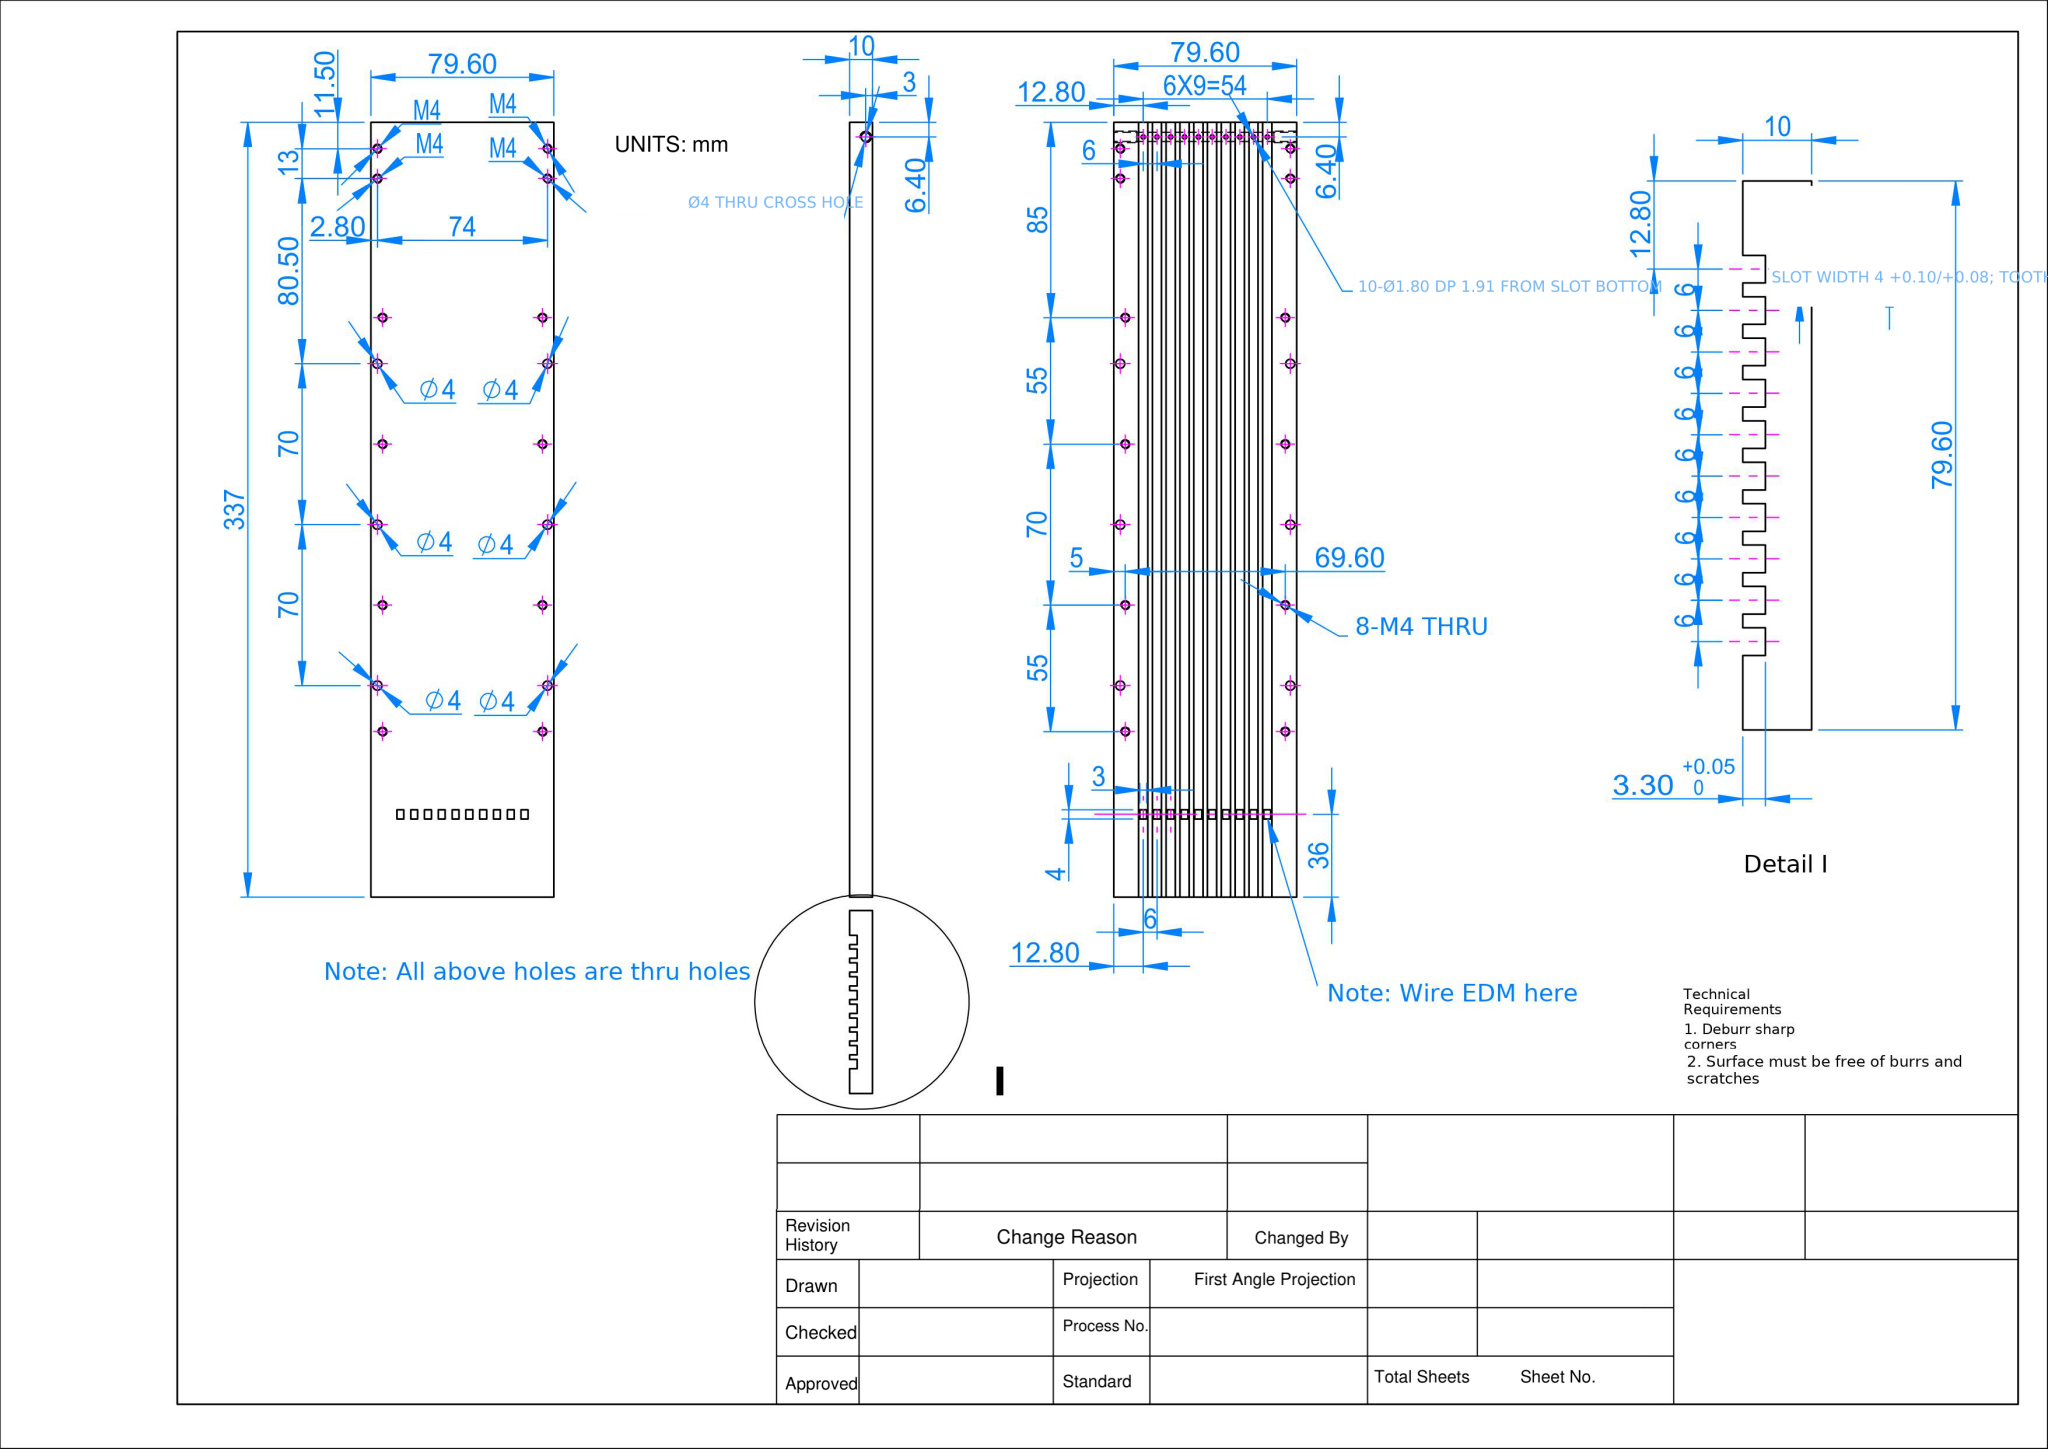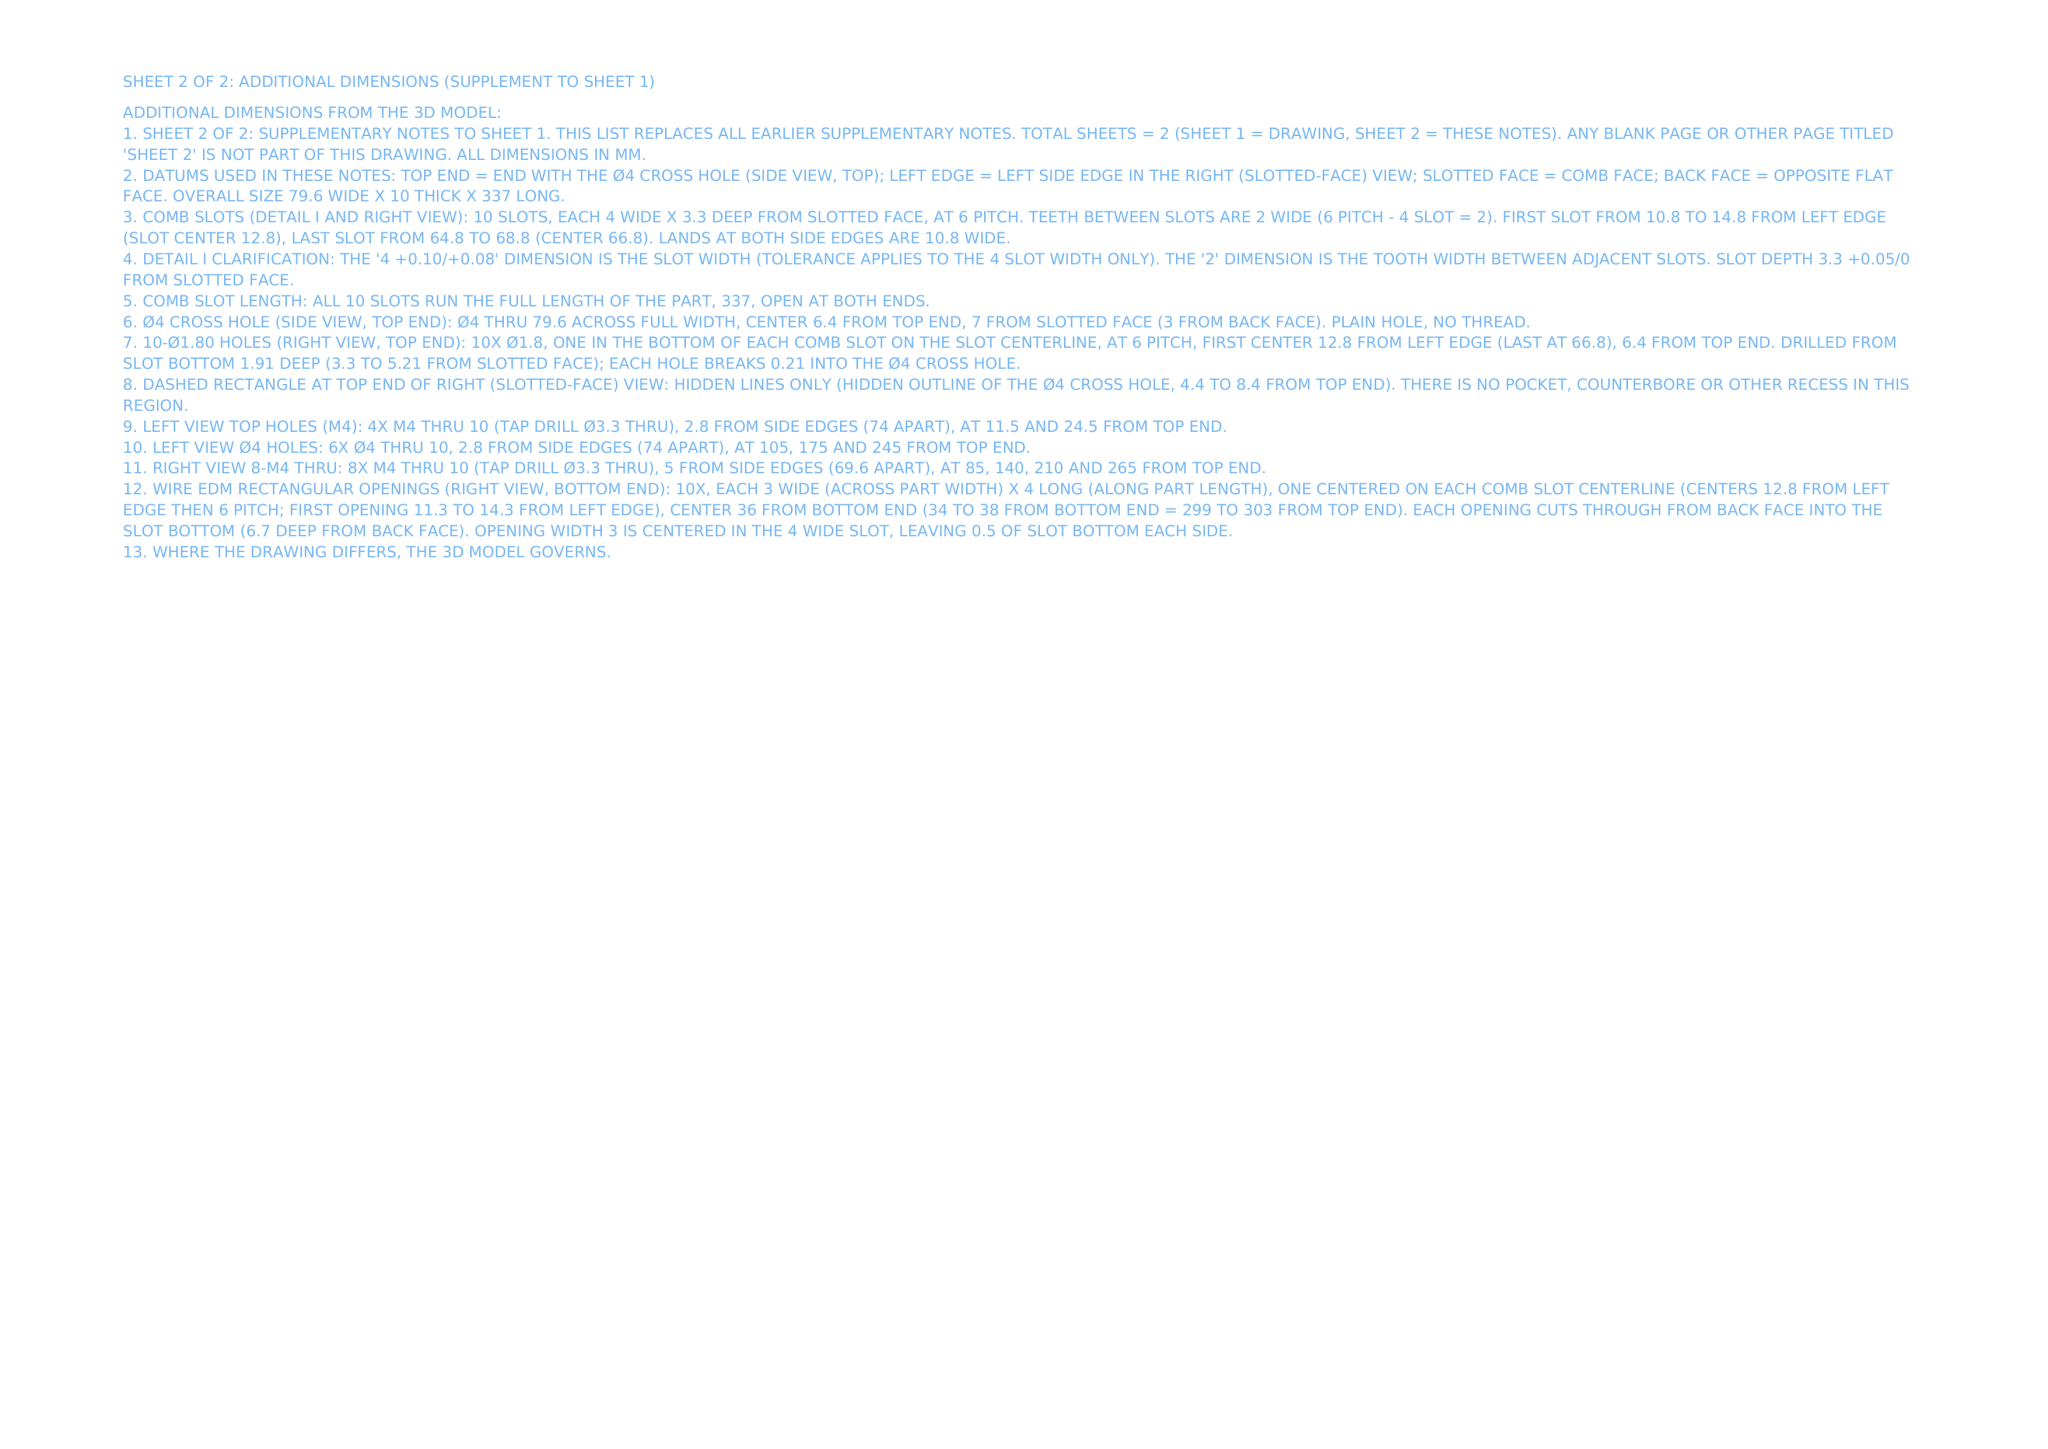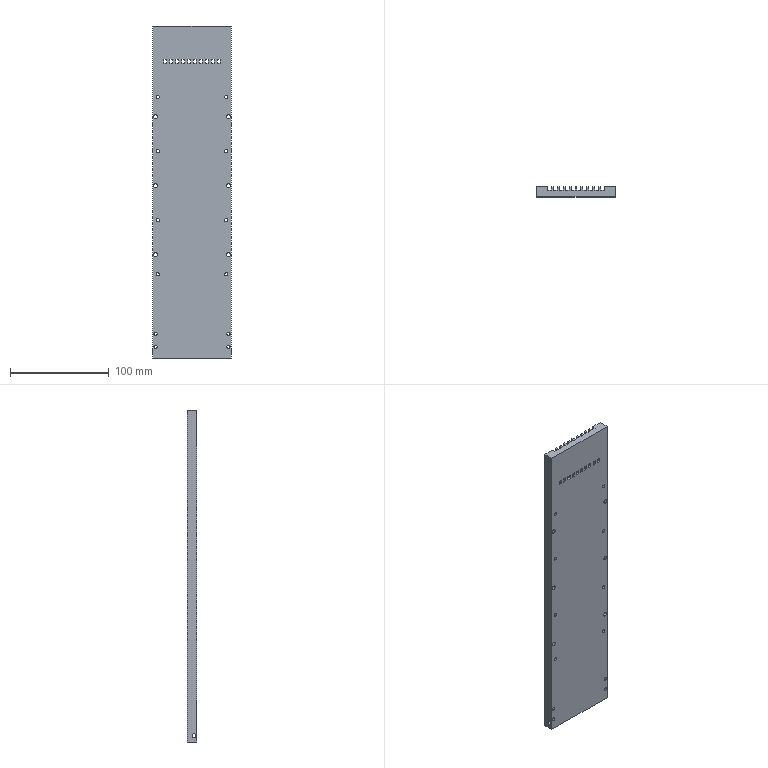Part | NX | mm | 1 solid | 144 faces | box 79.6 x 10 x 337 mm | volume 220139 mm3 | plane 86 | cylinder 58 | commonest cylinder face diameters 3.3 x24 1.8 x20 4 x14